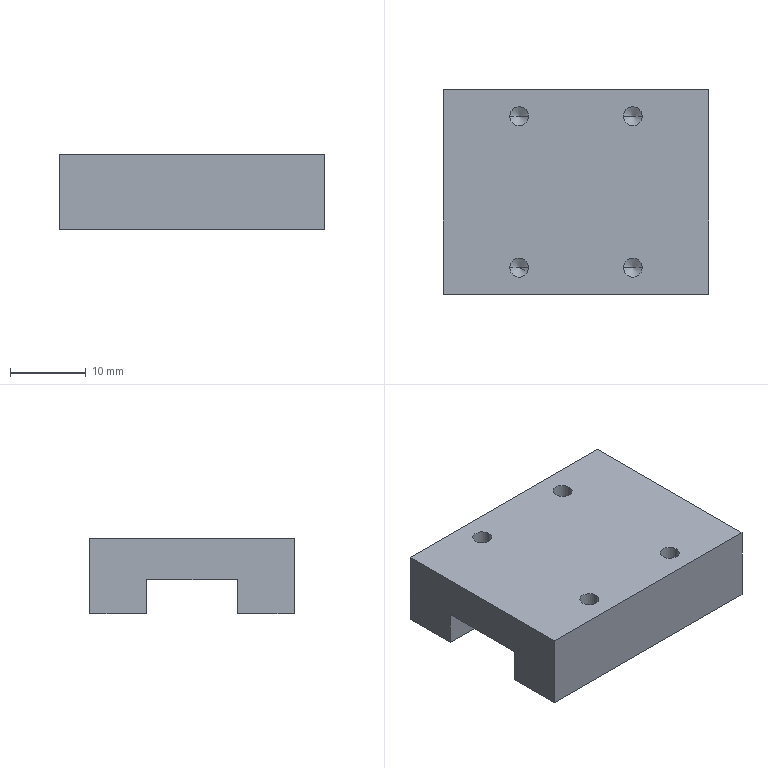Component | SolidWorks | TM12NNA-1-150-NA-Z0-1_TM12NN-1 | 1 solid | 26 faces | box 35 x 27 x 10 mm | volume 7388 mm3 | plane 10 | cylinder 8 | cone 8 | commonest cylinder face diameters 2.5 x8 | material 45
build123d program:
from build123d import *

# Parameters (mm, degrees)
SKETCH1_W           = 35
SKETCH1_H           = 27
BOSS_EXTRUDE1_DEPTH = 5
SKETCH2_W           = 4.5
SKETCH2_H           = 12
CUT_EXTRUDE1_DEPTH  = 38.845


with BuildPart() as part:
    # Sketch1 → Boss-Extrude1 (new, symmetric)
    with BuildSketch(Plane.XY):
        Rectangle(SKETCH1_W, SKETCH1_H)
    extrude(amount=BOSS_EXTRUDE1_DEPTH, both=True)

    # Sketch2 → Cut-Extrude1 (cut, through all)
    with BuildSketch(Plane(origin=(17.5, 0, 0), x_dir=(0, 0, -1), z_dir=(1, 0, 0))):
        with Locations((-2.75, 0)):
            Rectangle(SKETCH2_W, SKETCH2_H)
    extrude(amount=-CUT_EXTRUDE1_DEPTH, mode=Mode.SUBTRACT)

    # Sketch3 → M3 Tapped Hole1 (revolve, cut)
    with BuildSketch(Plane(origin=(7.5, -10, -5), x_dir=(0, 1, 0), z_dir=(1, 0, 0))):
        Polygon((0, 0), (0, 9.251), (1.25, 8.5), (1.25, 0), align=None)
    m3_tapped_hole1 = revolve(axis=Axis((7.5, -10, -11.35), (0, 0, 1)), mode=Mode.SUBTRACT)

    # Mirror1: M3 Tapped Hole1 across plane
    add(m3_tapped_hole1.mirror(Plane.ZX), mode=Mode.SUBTRACT)

    # Mirror2: M3 Tapped Hole1 across plane
    add(m3_tapped_hole1.mirror(Plane(origin=(0, 0, 0), x_dir=(0, 0, 1), z_dir=(1, 0, 0))), mode=Mode.SUBTRACT)

    # Mirror2 copy 1 sketch → Mirror2 copy 1 (revolve, cut)
    with BuildSketch(Plane(origin=(-7.5, 10, -5), x_dir=(0, -1, 0), z_dir=(-1, 0, 0))):
        Polygon((0, 0), (0, 9.251), (1.25, 8.5), (1.25, 0), align=None)
    revolve(axis=Axis((-7.5, 10, -11.35), (0, 0, 1)), mode=Mode.SUBTRACT)


solid = part.part

# Placed as in the assembly
solid = solid.moved(Location((171.3, 24, -67), (180, 0, 0)))
STEP:
#1=CARTESIAN_POINT('',(6.498,1.339,-2.776));
#2=VERTEX_POINT('',#1);
#3=CARTESIAN_POINT('',(6.4,1.339,-2.776));
#4=VERTEX_POINT('',#3);
#5=CARTESIAN_POINT('',(6.449,1.339,-2.776));
#6=DIRECTION('',(0.,0.,1.));
#7=DIRECTION('',(-1.,0.,0.));
#8=AXIS2_PLACEMENT_3D('',#5,#6,#7);
#9=CIRCLE('',#8,0.04921);
#10=EDGE_CURVE('',#2,#4,#9,.T.);
#11=ORIENTED_EDGE('',*,*,#10,.F.);
#12=CARTESIAN_POINT('',(6.498,1.339,-2.441));
#13=VERTEX_POINT('',#12);
#14=CARTESIAN_POINT('',(6.498,1.339,-2.441));
#15=DIRECTION('',(0.,0.,1.));
#16=VECTOR('',#15,39.37);
#17=LINE('',#14,#16);
#18=EDGE_CURVE('',#2,#13,#17,.T.);
#19=ORIENTED_EDGE('',*,*,#18,.T.);
#20=CARTESIAN_POINT('',(6.4,1.339,-2.441));
#21=VERTEX_POINT('',#20);
#22=CARTESIAN_POINT('',(6.449,1.339,-2.441));
#23=DIRECTION('',(0.,0.,1.));
#24=DIRECTION('',(-1.,0.,0.));
#25=AXIS2_PLACEMENT_3D('',#22,#23,#24);
#26=CIRCLE('',#25,0.04921);
#27=EDGE_CURVE('',#13,#21,#26,.T.);
#28=ORIENTED_EDGE('',*,*,#27,.T.);
#29=CARTESIAN_POINT('',(6.4,1.339,-2.441));
#30=DIRECTION('',(0.,0.,1.));
#31=VECTOR('',#30,39.37);
#32=LINE('',#29,#31);
#33=EDGE_CURVE('',#4,#21,#32,.T.);
#34=ORIENTED_EDGE('',*,*,#33,.F.);
#35=EDGE_LOOP('',(#11,#19,#28,#34));
#36=FACE_OUTER_BOUND('',#35,.T.);
#37=CARTESIAN_POINT('',(6.449,1.339,-2.441));
#38=DIRECTION('',(0.,0.,1.));
#39=DIRECTION('',(-1.,0.,0.));
#40=AXIS2_PLACEMENT_3D('',#37,#38,#39);
#41=CYLINDRICAL_SURFACE('',#40,0.04921);
#42=ADVANCED_FACE('',(#36),#41,.F.);
#43=CARTESIAN_POINT('',(6.449,1.339,-2.805));
#44=VERTEX_POINT('',#43);
#45=CARTESIAN_POINT('',(6.4,1.339,-2.776));
#46=DIRECTION('',(-0.8572,-0.,0.515));
#47=VECTOR('',#46,39.37);
#48=LINE('',#45,#47);
#49=EDGE_CURVE('',#44,#4,#48,.T.);
#50=ORIENTED_EDGE('',*,*,#49,.F.);
#51=CARTESIAN_POINT('',(6.498,1.339,-2.776));
#52=DIRECTION('',(0.8572,0.,0.515));
#53=VECTOR('',#52,39.37);
#54=LINE('',#51,#53);
#55=EDGE_CURVE('',#44,#2,#54,.T.);
#56=ORIENTED_EDGE('',*,*,#55,.T.);
#57=ORIENTED_EDGE('',*,*,#10,.T.);
#58=EDGE_LOOP('',(#50,#56,#57));
#59=FACE_OUTER_BOUND('',#58,.T.);
#60=CARTESIAN_POINT('',(6.449,1.339,-2.776));
#61=DIRECTION('',(0.,0.,1.));
#62=DIRECTION('',(-1.,0.,0.));
#63=AXIS2_PLACEMENT_3D('',#60,#61,#62);
#64=CONICAL_SURFACE('',#63,0.04921,1.03);
#65=ADVANCED_FACE('',(#59),#64,.F.);
#66=CARTESIAN_POINT('',(6.498,0.5512,-2.776));
#67=VERTEX_POINT('',#66);
#68=CARTESIAN_POINT('',(6.4,0.5512,-2.776));
#69=VERTEX_POINT('',#68);
#70=CARTESIAN_POINT('',(6.449,0.5512,-2.776));
#71=DIRECTION('',(0.,0.,1.));
#72=DIRECTION('',(-1.,0.,0.));
#73=AXIS2_PLACEMENT_3D('',#70,#71,#72);
#74=CIRCLE('',#73,0.04921);
#75=EDGE_CURVE('',#67,#69,#74,.T.);
#76=ORIENTED_EDGE('',*,*,#75,.F.);
#77=CARTESIAN_POINT('',(6.498,0.5512,-2.441));
#78=VERTEX_POINT('',#77);
#79=CARTESIAN_POINT('',(6.498,0.5512,-2.441));
#80=DIRECTION('',(0.,0.,1.));
#81=VECTOR('',#80,39.37);
#82=LINE('',#79,#81);
#83=EDGE_CURVE('',#67,#78,#82,.T.);
#84=ORIENTED_EDGE('',*,*,#83,.T.);
#85=CARTESIAN_POINT('',(6.4,0.5512,-2.441));
#86=VERTEX_POINT('',#85);
#87=CARTESIAN_POINT('',(6.449,0.5512,-2.441));
#88=DIRECTION('',(0.,0.,1.));
#89=DIRECTION('',(-1.,0.,0.));
#90=AXIS2_PLACEMENT_3D('',#87,#88,#89);
#91=CIRCLE('',#90,0.04921);
#92=EDGE_CURVE('',#78,#86,#91,.T.);
#93=ORIENTED_EDGE('',*,*,#92,.T.);
#94=CARTESIAN_POINT('',(6.4,0.5512,-2.441));
#95=DIRECTION('',(0.,0.,1.));
#96=VECTOR('',#95,39.37);
#97=LINE('',#94,#96);
#98=EDGE_CURVE('',#69,#86,#97,.T.);
#99=ORIENTED_EDGE('',*,*,#98,.F.);
#100=EDGE_LOOP('',(#76,#84,#93,#99));
#101=FACE_OUTER_BOUND('',#100,.T.);
#102=CARTESIAN_POINT('',(6.449,0.5512,-2.441));
#103=DIRECTION('',(0.,0.,1.));
#104=DIRECTION('',(-1.,0.,0.));
#105=AXIS2_PLACEMENT_3D('',#102,#103,#104);
#106=CYLINDRICAL_SURFACE('',#105,0.04921);
#107=ADVANCED_FACE('',(#101),#106,.F.);
#108=CARTESIAN_POINT('',(6.449,0.5512,-2.805));
#109=VERTEX_POINT('',#108);
#110=CARTESIAN_POINT('',(6.4,0.5512,-2.776));
#111=DIRECTION('',(-0.8572,-0.,0.515));
#112=VECTOR('',#111,39.37);
#113=LINE('',#110,#112);
#114=EDGE_CURVE('',#109,#69,#113,.T.);
#115=ORIENTED_EDGE('',*,*,#114,.F.);
#116=CARTESIAN_POINT('',(6.498,0.5512,-2.776));
#117=DIRECTION('',(0.8572,0.,0.515));
#118=VECTOR('',#117,39.37);
#119=LINE('',#116,#118);
#120=EDGE_CURVE('',#109,#67,#119,.T.);
#121=ORIENTED_EDGE('',*,*,#120,.T.);
#122=ORIENTED_EDGE('',*,*,#75,.T.);
#123=EDGE_LOOP('',(#115,#121,#122));
#124=FACE_OUTER_BOUND('',#123,.T.);
#125=CARTESIAN_POINT('',(6.449,0.5512,-2.776));
#126=DIRECTION('',(0.,0.,1.));
#127=DIRECTION('',(-1.,0.,0.));
#128=AXIS2_PLACEMENT_3D('',#125,#126,#127);
#129=CONICAL_SURFACE('',#128,0.04921,1.03);
#130=ADVANCED_FACE('',(#124),#129,.F.);
#131=CARTESIAN_POINT('',(7.089,0.5512,-2.776));
#132=VERTEX_POINT('',#131);
#133=CARTESIAN_POINT('',(6.99,0.5512,-2.776));
#134=VERTEX_POINT('',#133);
#135=CARTESIAN_POINT('',(7.039,0.5512,-2.776));
#136=DIRECTION('',(0.,0.,1.));
#137=DIRECTION('',(-1.,0.,0.));
#138=AXIS2_PLACEMENT_3D('',#135,#136,#137);
#139=CIRCLE('',#138,0.04921);
#140=EDGE_CURVE('',#132,#134,#139,.T.);
#141=ORIENTED_EDGE('',*,*,#140,.F.);
#142=CARTESIAN_POINT('',(7.089,0.5512,-2.441));
#143=VERTEX_POINT('',#142);
#144=CARTESIAN_POINT('',(7.089,0.5512,-2.441));
#145=DIRECTION('',(0.,0.,1.));
#146=VECTOR('',#145,39.37);
#147=LINE('',#144,#146);
#148=EDGE_CURVE('',#132,#143,#147,.T.);
#149=ORIENTED_EDGE('',*,*,#148,.T.);
#150=CARTESIAN_POINT('',(6.99,0.5512,-2.441));
#151=VERTEX_POINT('',#150);
#152=CARTESIAN_POINT('',(7.039,0.5512,-2.441));
#153=DIRECTION('',(0.,0.,1.));
#154=DIRECTION('',(-1.,0.,0.));
#155=AXIS2_PLACEMENT_3D('',#152,#153,#154);
#156=CIRCLE('',#155,0.04921);
#157=EDGE_CURVE('',#143,#151,#156,.T.);
#158=ORIENTED_EDGE('',*,*,#157,.T.);
#159=CARTESIAN_POINT('',(6.99,0.5512,-2.441));
#160=DIRECTION('',(0.,0.,1.));
#161=VECTOR('',#160,39.37);
#162=LINE('',#159,#161);
#163=EDGE_CURVE('',#134,#151,#162,.T.);
#164=ORIENTED_EDGE('',*,*,#163,.F.);
#165=EDGE_LOOP('',(#141,#149,#158,#164));
#166=FACE_OUTER_BOUND('',#165,.T.);
#167=CARTESIAN_POINT('',(7.039,0.5512,-2.441));
#168=DIRECTION('',(0.,0.,1.));
#169=DIRECTION('',(-1.,0.,0.));
#170=AXIS2_PLACEMENT_3D('',#167,#168,#169);
#171=CYLINDRICAL_SURFACE('',#170,0.04921);
#172=ADVANCED_FACE('',(#166),#171,.F.);
#173=CARTESIAN_POINT('',(7.039,0.5512,-2.805));
#174=VERTEX_POINT('',#173);
#175=CARTESIAN_POINT('',(6.99,0.5512,-2.776));
#176=DIRECTION('',(-0.8572,-0.,0.515));
#177=VECTOR('',#176,39.37);
#178=LINE('',#175,#177);
#179=EDGE_CURVE('',#174,#134,#178,.T.);
#180=ORIENTED_EDGE('',*,*,#179,.F.);
#181=CARTESIAN_POINT('',(7.089,0.5512,-2.776));
#182=DIRECTION('',(0.8572,0.,0.515));
#183=VECTOR('',#182,39.37);
#184=LINE('',#181,#183);
#185=EDGE_CURVE('',#174,#132,#184,.T.);
#186=ORIENTED_EDGE('',*,*,#185,.T.);
#187=ORIENTED_EDGE('',*,*,#140,.T.);
#188=EDGE_LOOP('',(#180,#186,#187));
#189=FACE_OUTER_BOUND('',#188,.T.);
#190=CARTESIAN_POINT('',(7.039,0.5512,-2.776));
#191=DIRECTION('',(0.,0.,1.));
#192=DIRECTION('',(-1.,0.,0.));
#193=AXIS2_PLACEMENT_3D('',#190,#191,#192);
#194=CONICAL_SURFACE('',#193,0.04921,1.03);
#195=ADVANCED_FACE('',(#189),#194,.F.);
#196=CARTESIAN_POINT('',(7.089,1.339,-2.776));
#197=VERTEX_POINT('',#196);
#198=CARTESIAN_POINT('',(6.99,1.339,-2.776));
#199=VERTEX_POINT('',#198);
#200=CARTESIAN_POINT('',(7.039,1.339,-2.776));
#201=DIRECTION('',(0.,0.,1.));
#202=DIRECTION('',(-1.,0.,0.));
#203=AXIS2_PLACEMENT_3D('',#200,#201,#202);
#204=CIRCLE('',#203,0.04921);
#205=EDGE_CURVE('',#197,#199,#204,.T.);
#206=ORIENTED_EDGE('',*,*,#205,.F.);
#207=CARTESIAN_POINT('',(7.089,1.339,-2.441));
#208=VERTEX_POINT('',#207);
#209=CARTESIAN_POINT('',(7.089,1.339,-2.441));
#210=DIRECTION('',(0.,0.,1.));
#211=VECTOR('',#210,39.37);
#212=LINE('',#209,#211);
#213=EDGE_CURVE('',#197,#208,#212,.T.);
#214=ORIENTED_EDGE('',*,*,#213,.T.);
#215=CARTESIAN_POINT('',(6.99,1.339,-2.441));
#216=VERTEX_POINT('',#215);
#217=CARTESIAN_POINT('',(7.039,1.339,-2.441));
#218=DIRECTION('',(0.,0.,1.));
#219=DIRECTION('',(-1.,0.,0.));
#220=AXIS2_PLACEMENT_3D('',#217,#218,#219);
#221=CIRCLE('',#220,0.04921);
#222=EDGE_CURVE('',#208,#216,#221,.T.);
#223=ORIENTED_EDGE('',*,*,#222,.T.);
#224=CARTESIAN_POINT('',(6.99,1.339,-2.441));
#225=DIRECTION('',(0.,0.,1.));
#226=VECTOR('',#225,39.37);
#227=LINE('',#224,#226);
#228=EDGE_CURVE('',#199,#216,#227,.T.);
#229=ORIENTED_EDGE('',*,*,#228,.F.);
#230=EDGE_LOOP('',(#206,#214,#223,#229));
#231=FACE_OUTER_BOUND('',#230,.T.);
#232=CARTESIAN_POINT('',(7.039,1.339,-2.441));
#233=DIRECTION('',(0.,0.,1.));
#234=DIRECTION('',(-1.,0.,0.));
#235=AXIS2_PLACEMENT_3D('',#232,#233,#234);
#236=CYLINDRICAL_SURFACE('',#235,0.04921);
#237=ADVANCED_FACE('',(#231),#236,.F.);
#238=CARTESIAN_POINT('',(7.039,1.339,-2.805));
#239=VERTEX_POINT('',#238);
#240=CARTESIAN_POINT('',(6.99,1.339,-2.776));
#241=DIRECTION('',(-0.8572,-0.,0.515));
#242=VECTOR('',#241,39.37);
#243=LINE('',#240,#242);
#244=EDGE_CURVE('',#239,#199,#243,.T.);
#245=ORIENTED_EDGE('',*,*,#244,.F.);
#246=CARTESIAN_POINT('',(7.089,1.339,-2.776));
#247=DIRECTION('',(0.8572,0.,0.515));
#248=VECTOR('',#247,39.37);
#249=LINE('',#246,#248);
#250=EDGE_CURVE('',#239,#197,#249,.T.);
#251=ORIENTED_EDGE('',*,*,#250,.T.);
#252=ORIENTED_EDGE('',*,*,#205,.T.);
#253=EDGE_LOOP('',(#245,#251,#252));
#254=FACE_OUTER_BOUND('',#253,.T.);
#255=CARTESIAN_POINT('',(7.039,1.339,-2.776));
#256=DIRECTION('',(0.,0.,1.));
#257=DIRECTION('',(-1.,0.,0.));
#258=AXIS2_PLACEMENT_3D('',#255,#256,#257);
#259=CONICAL_SURFACE('',#258,0.04921,1.03);
#260=ADVANCED_FACE('',(#254),#259,.F.);
#261=CARTESIAN_POINT('',(7.433,1.476,-2.835));
#262=VERTEX_POINT('',#261);
#263=CARTESIAN_POINT('',(7.433,1.181,-2.835));
#264=VERTEX_POINT('',#263);
#265=CARTESIAN_POINT('',(7.433,1.476,-2.835));
#266=DIRECTION('',(0.,-1.,0.));
#267=VECTOR('',#266,39.37);
#268=LINE('',#265,#267);
#269=EDGE_CURVE('',#262,#264,#268,.T.);
#270=ORIENTED_EDGE('',*,*,#269,.T.);
#271=CARTESIAN_POINT('',(6.055,1.181,-2.835));
#272=VERTEX_POINT('',#271);
#273=CARTESIAN_POINT('',(6.055,1.181,-2.835));
#274=DIRECTION('',(1.,0.,0.));
#275=VECTOR('',#274,39.37);
#276=LINE('',#273,#275);
#277=EDGE_CURVE('',#272,#264,#276,.T.);
#278=ORIENTED_EDGE('',*,*,#277,.F.);
#279=CARTESIAN_POINT('',(6.055,1.476,-2.835));
#280=VERTEX_POINT('',#279);
#281=CARTESIAN_POINT('',(6.055,1.476,-2.835));
#282=DIRECTION('',(-0.,1.,0.));
#283=VECTOR('',#282,39.37);
#284=LINE('',#281,#283);
#285=EDGE_CURVE('',#272,#280,#284,.T.);
#286=ORIENTED_EDGE('',*,*,#285,.T.);
#287=CARTESIAN_POINT('',(6.055,1.476,-2.835));
#288=DIRECTION('',(1.,0.,0.));
#289=VECTOR('',#288,39.37);
#290=LINE('',#287,#289);
#291=EDGE_CURVE('',#280,#262,#290,.T.);
#292=ORIENTED_EDGE('',*,*,#291,.T.);
#293=EDGE_LOOP('',(#270,#278,#286,#292));
#294=FACE_OUTER_BOUND('',#293,.T.);
#295=CARTESIAN_POINT('',(6.744,0.9449,-2.835));
#296=DIRECTION('',(0.,0.,1.));
#297=DIRECTION('',(-1.,-0.,0.));
#298=AXIS2_PLACEMENT_3D('',#295,#296,#297);
#299=PLANE('',#298);
#300=ADVANCED_FACE('',(#294),#299,.F.);
#301=CARTESIAN_POINT('',(7.433,1.181,-2.657));
#302=VERTEX_POINT('',#301);
#303=CARTESIAN_POINT('',(7.433,0.7087,-2.657));
#304=VERTEX_POINT('',#303);
#305=CARTESIAN_POINT('',(7.433,1.181,-2.657));
#306=DIRECTION('',(0.,-1.,0.));
#307=VECTOR('',#306,39.37);
#308=LINE('',#305,#307);
#309=EDGE_CURVE('',#302,#304,#308,.T.);
#310=ORIENTED_EDGE('',*,*,#309,.F.);
#311=CARTESIAN_POINT('',(7.433,1.181,-2.835));
#312=DIRECTION('',(0.,0.,1.));
#313=VECTOR('',#312,39.37);
#314=LINE('',#311,#313);
#315=EDGE_CURVE('',#264,#302,#314,.T.);
#316=ORIENTED_EDGE('',*,*,#315,.F.);
#317=ORIENTED_EDGE('',*,*,#269,.F.);
#318=CARTESIAN_POINT('',(7.433,1.476,-2.441));
#319=VERTEX_POINT('',#318);
#320=CARTESIAN_POINT('',(7.433,1.476,-2.835));
#321=DIRECTION('',(0.,0.,1.));
#322=VECTOR('',#321,39.37);
#323=LINE('',#320,#322);
#324=EDGE_CURVE('',#262,#319,#323,.T.);
#325=ORIENTED_EDGE('',*,*,#324,.T.);
#326=CARTESIAN_POINT('',(7.433,0.4134,-2.441));
#327=VERTEX_POINT('',#326);
#328=CARTESIAN_POINT('',(7.433,1.476,-2.441));
#329=DIRECTION('',(0.,-1.,0.));
#330=VECTOR('',#329,39.37);
#331=LINE('',#328,#330);
#332=EDGE_CURVE('',#319,#327,#331,.T.);
#333=ORIENTED_EDGE('',*,*,#332,.T.);
#334=CARTESIAN_POINT('',(7.433,0.4134,-2.835));
#335=VERTEX_POINT('',#334);
#336=CARTESIAN_POINT('',(7.433,0.4134,-2.835));
#337=DIRECTION('',(0.,0.,1.));
#338=VECTOR('',#337,39.37);
#339=LINE('',#336,#338);
#340=EDGE_CURVE('',#335,#327,#339,.T.);
#341=ORIENTED_EDGE('',*,*,#340,.F.);
#342=CARTESIAN_POINT('',(7.433,0.7087,-2.835));
#343=VERTEX_POINT('',#342);
#344=CARTESIAN_POINT('',(7.433,1.476,-2.835));
#345=DIRECTION('',(0.,-1.,0.));
#346=VECTOR('',#345,39.37);
#347=LINE('',#344,#346);
#348=EDGE_CURVE('',#343,#335,#347,.T.);
#349=ORIENTED_EDGE('',*,*,#348,.F.);
#350=CARTESIAN_POINT('',(7.433,0.7087,-2.835));
#351=DIRECTION('',(0.,0.,-1.));
#352=VECTOR('',#351,39.37);
#353=LINE('',#350,#352);
#354=EDGE_CURVE('',#304,#343,#353,.T.);
#355=ORIENTED_EDGE('',*,*,#354,.F.);
#356=EDGE_LOOP('',(#310,#316,#317,#325,#333,#341,#349,#355));
#357=FACE_OUTER_BOUND('',#356,.T.);
#358=CARTESIAN_POINT('',(7.433,1.476,-2.835));
#359=DIRECTION('',(-1.,-0.,0.));
#360=DIRECTION('',(0.,0.,-1.));
#361=AXIS2_PLACEMENT_3D('',#358,#359,#360);
#362=PLANE('',#361);
#363=ADVANCED_FACE('',(#357),#362,.F.);
#364=CARTESIAN_POINT('',(6.055,0.4134,-2.441));
#365=VERTEX_POINT('',#364);
#366=CARTESIAN_POINT('',(6.055,0.4134,-2.441));
#367=DIRECTION('',(-1.,-0.,0.));
#368=VECTOR('',#367,39.37);
#369=LINE('',#366,#368);
#370=EDGE_CURVE('',#327,#365,#369,.T.);
#371=ORIENTED_EDGE('',*,*,#370,.T.);
#372=CARTESIAN_POINT('',(6.055,0.4134,-2.835));
#373=VERTEX_POINT('',#372);
#374=CARTESIAN_POINT('',(6.055,0.4134,-2.835));
#375=DIRECTION('',(0.,0.,1.));
#376=VECTOR('',#375,39.37);
#377=LINE('',#374,#376);
#378=EDGE_CURVE('',#373,#365,#377,.T.);
#379=ORIENTED_EDGE('',*,*,#378,.F.);
#380=CARTESIAN_POINT('',(6.055,0.4134,-2.835));
#381=DIRECTION('',(-1.,-0.,0.));
#382=VECTOR('',#381,39.37);
#383=LINE('',#380,#382);
#384=EDGE_CURVE('',#335,#373,#383,.T.);
#385=ORIENTED_EDGE('',*,*,#384,.F.);
#386=ORIENTED_EDGE('',*,*,#340,.T.);
#387=EDGE_LOOP('',(#371,#379,#385,#386));
#388=FACE_OUTER_BOUND('',#387,.T.);
#389=CARTESIAN_POINT('',(6.055,0.4134,-2.835));
#390=DIRECTION('',(-0.,1.,0.));
#391=DIRECTION('',(0.,0.,1.));
#392=AXIS2_PLACEMENT_3D('',#389,#390,#391);
#393=PLANE('',#392);
#394=ADVANCED_FACE('',(#388),#393,.F.);
#395=ORIENTED_EDGE('',*,*,#285,.F.);
#396=CARTESIAN_POINT('',(6.055,1.181,-2.657));
#397=VERTEX_POINT('',#396);
#398=CARTESIAN_POINT('',(6.055,1.181,-2.835));
#399=DIRECTION('',(0.,0.,1.));
#400=VECTOR('',#399,39.37);
#401=LINE('',#398,#400);
#402=EDGE_CURVE('',#272,#397,#401,.T.);
#403=ORIENTED_EDGE('',*,*,#402,.T.);
#404=CARTESIAN_POINT('',(6.055,0.7087,-2.657));
#405=VERTEX_POINT('',#404);
#406=CARTESIAN_POINT('',(6.055,1.181,-2.657));
#407=DIRECTION('',(0.,-1.,0.));
#408=VECTOR('',#407,39.37);
#409=LINE('',#406,#408);
#410=EDGE_CURVE('',#397,#405,#409,.T.);
#411=ORIENTED_EDGE('',*,*,#410,.T.);
#412=CARTESIAN_POINT('',(6.055,0.7087,-2.835));
#413=VERTEX_POINT('',#412);
#414=CARTESIAN_POINT('',(6.055,0.7087,-2.835));
#415=DIRECTION('',(0.,0.,-1.));
#416=VECTOR('',#415,39.37);
#417=LINE('',#414,#416);
#418=EDGE_CURVE('',#405,#413,#417,.T.);
#419=ORIENTED_EDGE('',*,*,#418,.T.);
#420=CARTESIAN_POINT('',(6.055,1.476,-2.835));
#421=DIRECTION('',(-0.,1.,0.));
#422=VECTOR('',#421,39.37);
#423=LINE('',#420,#422);
#424=EDGE_CURVE('',#373,#413,#423,.T.);
#425=ORIENTED_EDGE('',*,*,#424,.F.);
#426=ORIENTED_EDGE('',*,*,#378,.T.);
#427=CARTESIAN_POINT('',(6.055,1.476,-2.441));
#428=VERTEX_POINT('',#427);
#429=CARTESIAN_POINT('',(6.055,1.476,-2.441));
#430=DIRECTION('',(-0.,1.,0.));
#431=VECTOR('',#430,39.37);
#432=LINE('',#429,#431);
#433=EDGE_CURVE('',#365,#428,#432,.T.);
#434=ORIENTED_EDGE('',*,*,#433,.T.);
#435=CARTESIAN_POINT('',(6.055,1.476,-2.835));
#436=DIRECTION('',(0.,0.,1.));
#437=VECTOR('',#436,39.37);
#438=LINE('',#435,#437);
#439=EDGE_CURVE('',#280,#428,#438,.T.);
#440=ORIENTED_EDGE('',*,*,#439,.F.);
#441=EDGE_LOOP('',(#395,#403,#411,#419,#425,#426,#434,#440));
#442=FACE_OUTER_BOUND('',#441,.T.);
#443=CARTESIAN_POINT('',(6.055,1.476,-2.835));
#444=DIRECTION('',(1.,0.,0.));
#445=DIRECTION('',(0.,0.,1.));
#446=AXIS2_PLACEMENT_3D('',#443,#444,#445);
#447=PLANE('',#446);
#448=ADVANCED_FACE('',(#442),#447,.F.);
#449=CARTESIAN_POINT('',(6.055,1.476,-2.441));
#450=DIRECTION('',(1.,0.,0.));
#451=VECTOR('',#450,39.37);
#452=LINE('',#449,#451);
#453=EDGE_CURVE('',#428,#319,#452,.T.);
#454=ORIENTED_EDGE('',*,*,#453,.T.);
#455=ORIENTED_EDGE('',*,*,#324,.F.);
#456=ORIENTED_EDGE('',*,*,#291,.F.);
#457=ORIENTED_EDGE('',*,*,#439,.T.);
#458=EDGE_LOOP('',(#454,#455,#456,#457));
#459=FACE_OUTER_BOUND('',#458,.T.);
#460=CARTESIAN_POINT('',(6.055,1.476,-2.835));
#461=DIRECTION('',(0.,-1.,0.));
#462=DIRECTION('',(0.,0.,-1.));
#463=AXIS2_PLACEMENT_3D('',#460,#461,#462);
#464=PLANE('',#463);
#465=ADVANCED_FACE('',(#459),#464,.F.);
#466=ORIENTED_EDGE('',*,*,#424,.T.);
#467=CARTESIAN_POINT('',(6.055,0.7087,-2.835));
#468=DIRECTION('',(1.,0.,0.));
#469=VECTOR('',#468,39.37);
#470=LINE('',#467,#469);
#471=EDGE_CURVE('',#413,#343,#470,.T.);
#472=ORIENTED_EDGE('',*,*,#471,.T.);
#473=ORIENTED_EDGE('',*,*,#348,.T.);
#474=ORIENTED_EDGE('',*,*,#384,.T.);
#475=EDGE_LOOP('',(#466,#472,#473,#474));
#476=FACE_OUTER_BOUND('',#475,.T.);
#477=CARTESIAN_POINT('',(6.744,0.9449,-2.835));
#478=DIRECTION('',(0.,0.,1.));
#479=DIRECTION('',(-1.,-0.,0.));
#480=AXIS2_PLACEMENT_3D('',#477,#478,#479);
#481=PLANE('',#480);
#482=ADVANCED_FACE('',(#476),#481,.F.);
#483=CARTESIAN_POINT('',(6.449,1.339,-2.441));
#484=DIRECTION('',(0.,0.,1.));
#485=DIRECTION('',(-1.,0.,0.));
#486=AXIS2_PLACEMENT_3D('',#483,#484,#485);
#487=CIRCLE('',#486,0.04921);
#488=EDGE_CURVE('',#21,#13,#487,.T.);
#489=ORIENTED_EDGE('',*,*,#488,.F.);
#490=ORIENTED_EDGE('',*,*,#27,.F.);
#491=EDGE_LOOP('',(#489,#490));
#492=FACE_BOUND('',#491,.T.);
#493=CARTESIAN_POINT('',(6.449,0.5512,-2.441));
#494=DIRECTION('',(0.,0.,1.));
#495=DIRECTION('',(-1.,0.,0.));
#496=AXIS2_PLACEMENT_3D('',#493,#494,#495);
#497=CIRCLE('',#496,0.04921);
#498=EDGE_CURVE('',#86,#78,#497,.T.);
#499=ORIENTED_EDGE('',*,*,#498,.F.);
#500=ORIENTED_EDGE('',*,*,#92,.F.);
#501=EDGE_LOOP('',(#499,#500));
#502=FACE_BOUND('',#501,.T.);
#503=CARTESIAN_POINT('',(7.039,0.5512,-2.441));
#504=DIRECTION('',(0.,0.,1.));
#505=DIRECTION('',(-1.,0.,0.));
#506=AXIS2_PLACEMENT_3D('',#503,#504,#505);
#507=CIRCLE('',#506,0.04921);
#508=EDGE_CURVE('',#151,#143,#507,.T.);
#509=ORIENTED_EDGE('',*,*,#508,.F.);
#510=ORIENTED_EDGE('',*,*,#157,.F.);
#511=EDGE_LOOP('',(#509,#510));
#512=FACE_BOUND('',#511,.T.);
#513=CARTESIAN_POINT('',(7.039,1.339,-2.441));
#514=DIRECTION('',(0.,0.,1.));
#515=DIRECTION('',(-1.,0.,0.));
#516=AXIS2_PLACEMENT_3D('',#513,#514,#515);
#517=CIRCLE('',#516,0.04921);
#518=EDGE_CURVE('',#216,#208,#517,.T.);
#519=ORIENTED_EDGE('',*,*,#518,.F.);
#520=ORIENTED_EDGE('',*,*,#222,.F.);
#521=EDGE_LOOP('',(#519,#520));
#522=FACE_BOUND('',#521,.T.);
#523=ORIENTED_EDGE('',*,*,#332,.F.);
#524=ORIENTED_EDGE('',*,*,#453,.F.);
#525=ORIENTED_EDGE('',*,*,#433,.F.);
#526=ORIENTED_EDGE('',*,*,#370,.F.);
#527=EDGE_LOOP('',(#523,#524,#525,#526));
#528=FACE_OUTER_BOUND('',#527,.T.);
#529=CARTESIAN_POINT('',(6.744,0.9449,-2.441));
#530=DIRECTION('',(0.,0.,1.));
#531=DIRECTION('',(-1.,-0.,0.));
#532=AXIS2_PLACEMENT_3D('',#529,#530,#531);
#533=PLANE('',#532);
#534=ADVANCED_FACE('',(#492,#502,#512,#522,#528),#533,.T.);
#535=ORIENTED_EDGE('',*,*,#309,.T.);
#536=CARTESIAN_POINT('',(6.055,0.7087,-2.657));
#537=DIRECTION('',(1.,0.,0.));
#538=VECTOR('',#537,39.37);
#539=LINE('',#536,#538);
#540=EDGE_CURVE('',#405,#304,#539,.T.);
#541=ORIENTED_EDGE('',*,*,#540,.F.);
#542=ORIENTED_EDGE('',*,*,#410,.F.);
#543=CARTESIAN_POINT('',(6.055,1.181,-2.657));
#544=DIRECTION('',(1.,0.,0.));
#545=VECTOR('',#544,39.37);
#546=LINE('',#543,#545);
#547=EDGE_CURVE('',#397,#302,#546,.T.);
#548=ORIENTED_EDGE('',*,*,#547,.T.);
#549=EDGE_LOOP('',(#535,#541,#542,#548));
#550=FACE_OUTER_BOUND('',#549,.T.);
#551=CARTESIAN_POINT('',(6.055,1.181,-2.657));
#552=DIRECTION('',(0.,0.,1.));
#553=DIRECTION('',(-1.,-0.,0.));
#554=AXIS2_PLACEMENT_3D('',#551,#552,#553);
#555=PLANE('',#554);
#556=ADVANCED_FACE('',(#550),#555,.F.);
#557=ORIENTED_EDGE('',*,*,#315,.T.);
#558=ORIENTED_EDGE('',*,*,#547,.F.);
#559=ORIENTED_EDGE('',*,*,#402,.F.);
#560=ORIENTED_EDGE('',*,*,#277,.T.);
#561=EDGE_LOOP('',(#557,#558,#559,#560));
#562=FACE_OUTER_BOUND('',#561,.T.);
#563=CARTESIAN_POINT('',(6.055,1.181,-2.835));
#564=DIRECTION('',(-0.,1.,0.));
#565=DIRECTION('',(0.,0.,1.));
#566=AXIS2_PLACEMENT_3D('',#563,#564,#565);
#567=PLANE('',#566);
#568=ADVANCED_FACE('',(#562),#567,.F.);
#569=ORIENTED_EDGE('',*,*,#354,.T.);
#570=ORIENTED_EDGE('',*,*,#471,.F.);
#571=ORIENTED_EDGE('',*,*,#418,.F.);
#572=ORIENTED_EDGE('',*,*,#540,.T.);
#573=EDGE_LOOP('',(#569,#570,#571,#572));
#574=FACE_OUTER_BOUND('',#573,.T.);
#575=CARTESIAN_POINT('',(6.055,0.7087,-2.835));
#576=DIRECTION('',(0.,-1.,0.));
#577=DIRECTION('',(0.,0.,-1.));
#578=AXIS2_PLACEMENT_3D('',#575,#576,#577);
#579=PLANE('',#578);
#580=ADVANCED_FACE('',(#574),#579,.F.);
#581=ORIENTED_EDGE('',*,*,#250,.F.);
#582=ORIENTED_EDGE('',*,*,#244,.T.);
#583=CARTESIAN_POINT('',(7.039,1.339,-2.776));
#584=DIRECTION('',(0.,0.,1.));
#585=DIRECTION('',(-1.,0.,0.));
#586=AXIS2_PLACEMENT_3D('',#583,#584,#585);
#587=CIRCLE('',#586,0.04921);
#588=EDGE_CURVE('',#199,#197,#587,.T.);
#589=ORIENTED_EDGE('',*,*,#588,.T.);
#590=EDGE_LOOP('',(#581,#582,#589));
#591=FACE_OUTER_BOUND('',#590,.T.);
#592=CARTESIAN_POINT('',(7.039,1.339,-2.776));
#593=DIRECTION('',(0.,0.,1.));
#594=DIRECTION('',(-1.,0.,0.));
#595=AXIS2_PLACEMENT_3D('',#592,#593,#594);
#596=CONICAL_SURFACE('',#595,0.04921,1.03);
#597=ADVANCED_FACE('',(#591),#596,.F.);
#598=ORIENTED_EDGE('',*,*,#213,.F.);
#599=ORIENTED_EDGE('',*,*,#588,.F.);
#600=ORIENTED_EDGE('',*,*,#228,.T.);
#601=ORIENTED_EDGE('',*,*,#518,.T.);
#602=EDGE_LOOP('',(#598,#599,#600,#601));
#603=FACE_OUTER_BOUND('',#602,.T.);
#604=CARTESIAN_POINT('',(7.039,1.339,-2.441));
#605=DIRECTION('',(0.,0.,1.));
#606=DIRECTION('',(-1.,0.,0.));
#607=AXIS2_PLACEMENT_3D('',#604,#605,#606);
#608=CYLINDRICAL_SURFACE('',#607,0.04921);
#609=ADVANCED_FACE('',(#603),#608,.F.);
#610=ORIENTED_EDGE('',*,*,#185,.F.);
#611=ORIENTED_EDGE('',*,*,#179,.T.);
#612=CARTESIAN_POINT('',(7.039,0.5512,-2.776));
#613=DIRECTION('',(0.,0.,1.));
#614=DIRECTION('',(-1.,0.,0.));
#615=AXIS2_PLACEMENT_3D('',#612,#613,#614);
#616=CIRCLE('',#615,0.04921);
#617=EDGE_CURVE('',#134,#132,#616,.T.);
#618=ORIENTED_EDGE('',*,*,#617,.T.);
#619=EDGE_LOOP('',(#610,#611,#618));
#620=FACE_OUTER_BOUND('',#619,.T.);
#621=CARTESIAN_POINT('',(7.039,0.5512,-2.776));
#622=DIRECTION('',(0.,0.,1.));
#623=DIRECTION('',(-1.,0.,0.));
#624=AXIS2_PLACEMENT_3D('',#621,#622,#623);
#625=CONICAL_SURFACE('',#624,0.04921,1.03);
#626=ADVANCED_FACE('',(#620),#625,.F.);
#627=ORIENTED_EDGE('',*,*,#148,.F.);
#628=ORIENTED_EDGE('',*,*,#617,.F.);
#629=ORIENTED_EDGE('',*,*,#163,.T.);
#630=ORIENTED_EDGE('',*,*,#508,.T.);
#631=EDGE_LOOP('',(#627,#628,#629,#630));
#632=FACE_OUTER_BOUND('',#631,.T.);
#633=CARTESIAN_POINT('',(7.039,0.5512,-2.441));
#634=DIRECTION('',(0.,0.,1.));
#635=DIRECTION('',(-1.,0.,0.));
#636=AXIS2_PLACEMENT_3D('',#633,#634,#635);
#637=CYLINDRICAL_SURFACE('',#636,0.04921);
#638=ADVANCED_FACE('',(#632),#637,.F.);
#639=ORIENTED_EDGE('',*,*,#120,.F.);
#640=ORIENTED_EDGE('',*,*,#114,.T.);
#641=CARTESIAN_POINT('',(6.449,0.5512,-2.776));
#642=DIRECTION('',(0.,0.,1.));
#643=DIRECTION('',(-1.,0.,0.));
#644=AXIS2_PLACEMENT_3D('',#641,#642,#643);
#645=CIRCLE('',#644,0.04921);
#646=EDGE_CURVE('',#69,#67,#645,.T.);
#647=ORIENTED_EDGE('',*,*,#646,.T.);
#648=EDGE_LOOP('',(#639,#640,#647));
#649=FACE_OUTER_BOUND('',#648,.T.);
#650=CARTESIAN_POINT('',(6.449,0.5512,-2.776));
#651=DIRECTION('',(0.,0.,1.));
#652=DIRECTION('',(-1.,0.,0.));
#653=AXIS2_PLACEMENT_3D('',#650,#651,#652);
#654=CONICAL_SURFACE('',#653,0.04921,1.03);
#655=ADVANCED_FACE('',(#649),#654,.F.);
#656=ORIENTED_EDGE('',*,*,#83,.F.);
#657=ORIENTED_EDGE('',*,*,#646,.F.);
#658=ORIENTED_EDGE('',*,*,#98,.T.);
#659=ORIENTED_EDGE('',*,*,#498,.T.);
#660=EDGE_LOOP('',(#656,#657,#658,#659));
#661=FACE_OUTER_BOUND('',#660,.T.);
#662=CARTESIAN_POINT('',(6.449,0.5512,-2.441));
#663=DIRECTION('',(0.,0.,1.));
#664=DIRECTION('',(-1.,0.,0.));
#665=AXIS2_PLACEMENT_3D('',#662,#663,#664);
#666=CYLINDRICAL_SURFACE('',#665,0.04921);
#667=ADVANCED_FACE('',(#661),#666,.F.);
#668=ORIENTED_EDGE('',*,*,#55,.F.);
#669=ORIENTED_EDGE('',*,*,#49,.T.);
#670=CARTESIAN_POINT('',(6.449,1.339,-2.776));
#671=DIRECTION('',(0.,0.,1.));
#672=DIRECTION('',(-1.,0.,0.));
#673=AXIS2_PLACEMENT_3D('',#670,#671,#672);
#674=CIRCLE('',#673,0.04921);
#675=EDGE_CURVE('',#4,#2,#674,.T.);
#676=ORIENTED_EDGE('',*,*,#675,.T.);
#677=EDGE_LOOP('',(#668,#669,#676));
#678=FACE_OUTER_BOUND('',#677,.T.);
#679=CARTESIAN_POINT('',(6.449,1.339,-2.776));
#680=DIRECTION('',(0.,0.,1.));
#681=DIRECTION('',(-1.,0.,0.));
#682=AXIS2_PLACEMENT_3D('',#679,#680,#681);
#683=CONICAL_SURFACE('',#682,0.04921,1.03);
#684=ADVANCED_FACE('',(#678),#683,.F.);
#685=ORIENTED_EDGE('',*,*,#18,.F.);
#686=ORIENTED_EDGE('',*,*,#675,.F.);
#687=ORIENTED_EDGE('',*,*,#33,.T.);
#688=ORIENTED_EDGE('',*,*,#488,.T.);
#689=EDGE_LOOP('',(#685,#686,#687,#688));
#690=FACE_OUTER_BOUND('',#689,.T.);
#691=CARTESIAN_POINT('',(6.449,1.339,-2.441));
#692=DIRECTION('',(0.,0.,1.));
#693=DIRECTION('',(-1.,0.,0.));
#694=AXIS2_PLACEMENT_3D('',#691,#692,#693);
#695=CYLINDRICAL_SURFACE('',#694,0.04921);
#696=ADVANCED_FACE('',(#690),#695,.F.);
#697=CLOSED_SHELL('',(#42,#65,#107,#130,#172,#195,#237,#260,#300,#363,#394,#448,#465,#482,#534,#556,#568,#580,#597,#609,#626,#638,#655,#667,#684,#696));
#698=MANIFOLD_SOLID_BREP('',#697);
#699=CARTESIAN_POINT('',(0.,0.,0.));
#700=DIRECTION('',(0.,0.,1.));
#701=DIRECTION('',(1.,0.,0.));
#702=AXIS2_PLACEMENT_3D('',#699,#700,#701);
#703=(LENGTH_UNIT()NAMED_UNIT(*)SI_UNIT($,.METRE.));
#704=LENGTH_MEASURE_WITH_UNIT(LENGTH_MEASURE(0.0254),#703);
#705=DIMENSIONAL_EXPONENTS(1.,0.,0.,0.,0.,0.,0.);
#706=(CONVERSION_BASED_UNIT('',#704)LENGTH_UNIT()NAMED_UNIT(#705));
#707=UNCERTAINTY_MEASURE_WITH_UNIT(LENGTH_MEASURE(0.00001),#706,'','');
#708=(NAMED_UNIT(*)PLANE_ANGLE_UNIT()SI_UNIT($,.RADIAN.));
#709=(NAMED_UNIT(*)SI_UNIT($,.STERADIAN.)SOLID_ANGLE_UNIT());
#710=(GEOMETRIC_REPRESENTATION_CONTEXT(3)GLOBAL_UNCERTAINTY_ASSIGNED_CONTEXT((#707))GLOBAL_UNIT_ASSIGNED_CONTEXT((#706,#708,#709))REPRESENTATION_CONTEXT('',''));
#711=ADVANCED_BREP_SHAPE_REPRESENTATION('',(#698,#702),#710);
#712=COLOUR_RGB('',0.7922,0.8196,0.9333);
#713=FILL_AREA_STYLE_COLOUR('',#712);
#714=FILL_AREA_STYLE('',(#713));
#715=SURFACE_STYLE_FILL_AREA(#714);
#716=SURFACE_SIDE_STYLE('',(#715));
#717=SURFACE_STYLE_USAGE(.BOTH.,#716);
#718=PRESENTATION_STYLE_ASSIGNMENT((#717));
#719=STYLED_ITEM('',(#718),#698);
#720=PRESENTATION_LAYER_ASSIGNMENT('','',(#719));
#721=(LENGTH_UNIT()NAMED_UNIT(*)SI_UNIT($,.METRE.));
#722=LENGTH_MEASURE_WITH_UNIT(LENGTH_MEASURE(0.0254),#721);
#723=DIMENSIONAL_EXPONENTS(1.,0.,0.,0.,0.,0.,0.);
#724=(CONVERSION_BASED_UNIT('',#722)LENGTH_UNIT()NAMED_UNIT(#723));
#725=UNCERTAINTY_MEASURE_WITH_UNIT(LENGTH_MEASURE(0.00001),#724,'','');
#726=(NAMED_UNIT(*)PLANE_ANGLE_UNIT()SI_UNIT($,.RADIAN.));
#727=(NAMED_UNIT(*)SI_UNIT($,.STERADIAN.)SOLID_ANGLE_UNIT());
#728=(GEOMETRIC_REPRESENTATION_CONTEXT(3)GLOBAL_UNCERTAINTY_ASSIGNED_CONTEXT((#725))GLOBAL_UNIT_ASSIGNED_CONTEXT((#724,#726,#727))REPRESENTATION_CONTEXT('',''));
#729=MECHANICAL_DESIGN_GEOMETRIC_PRESENTATION_REPRESENTATION('',(#719),#728);